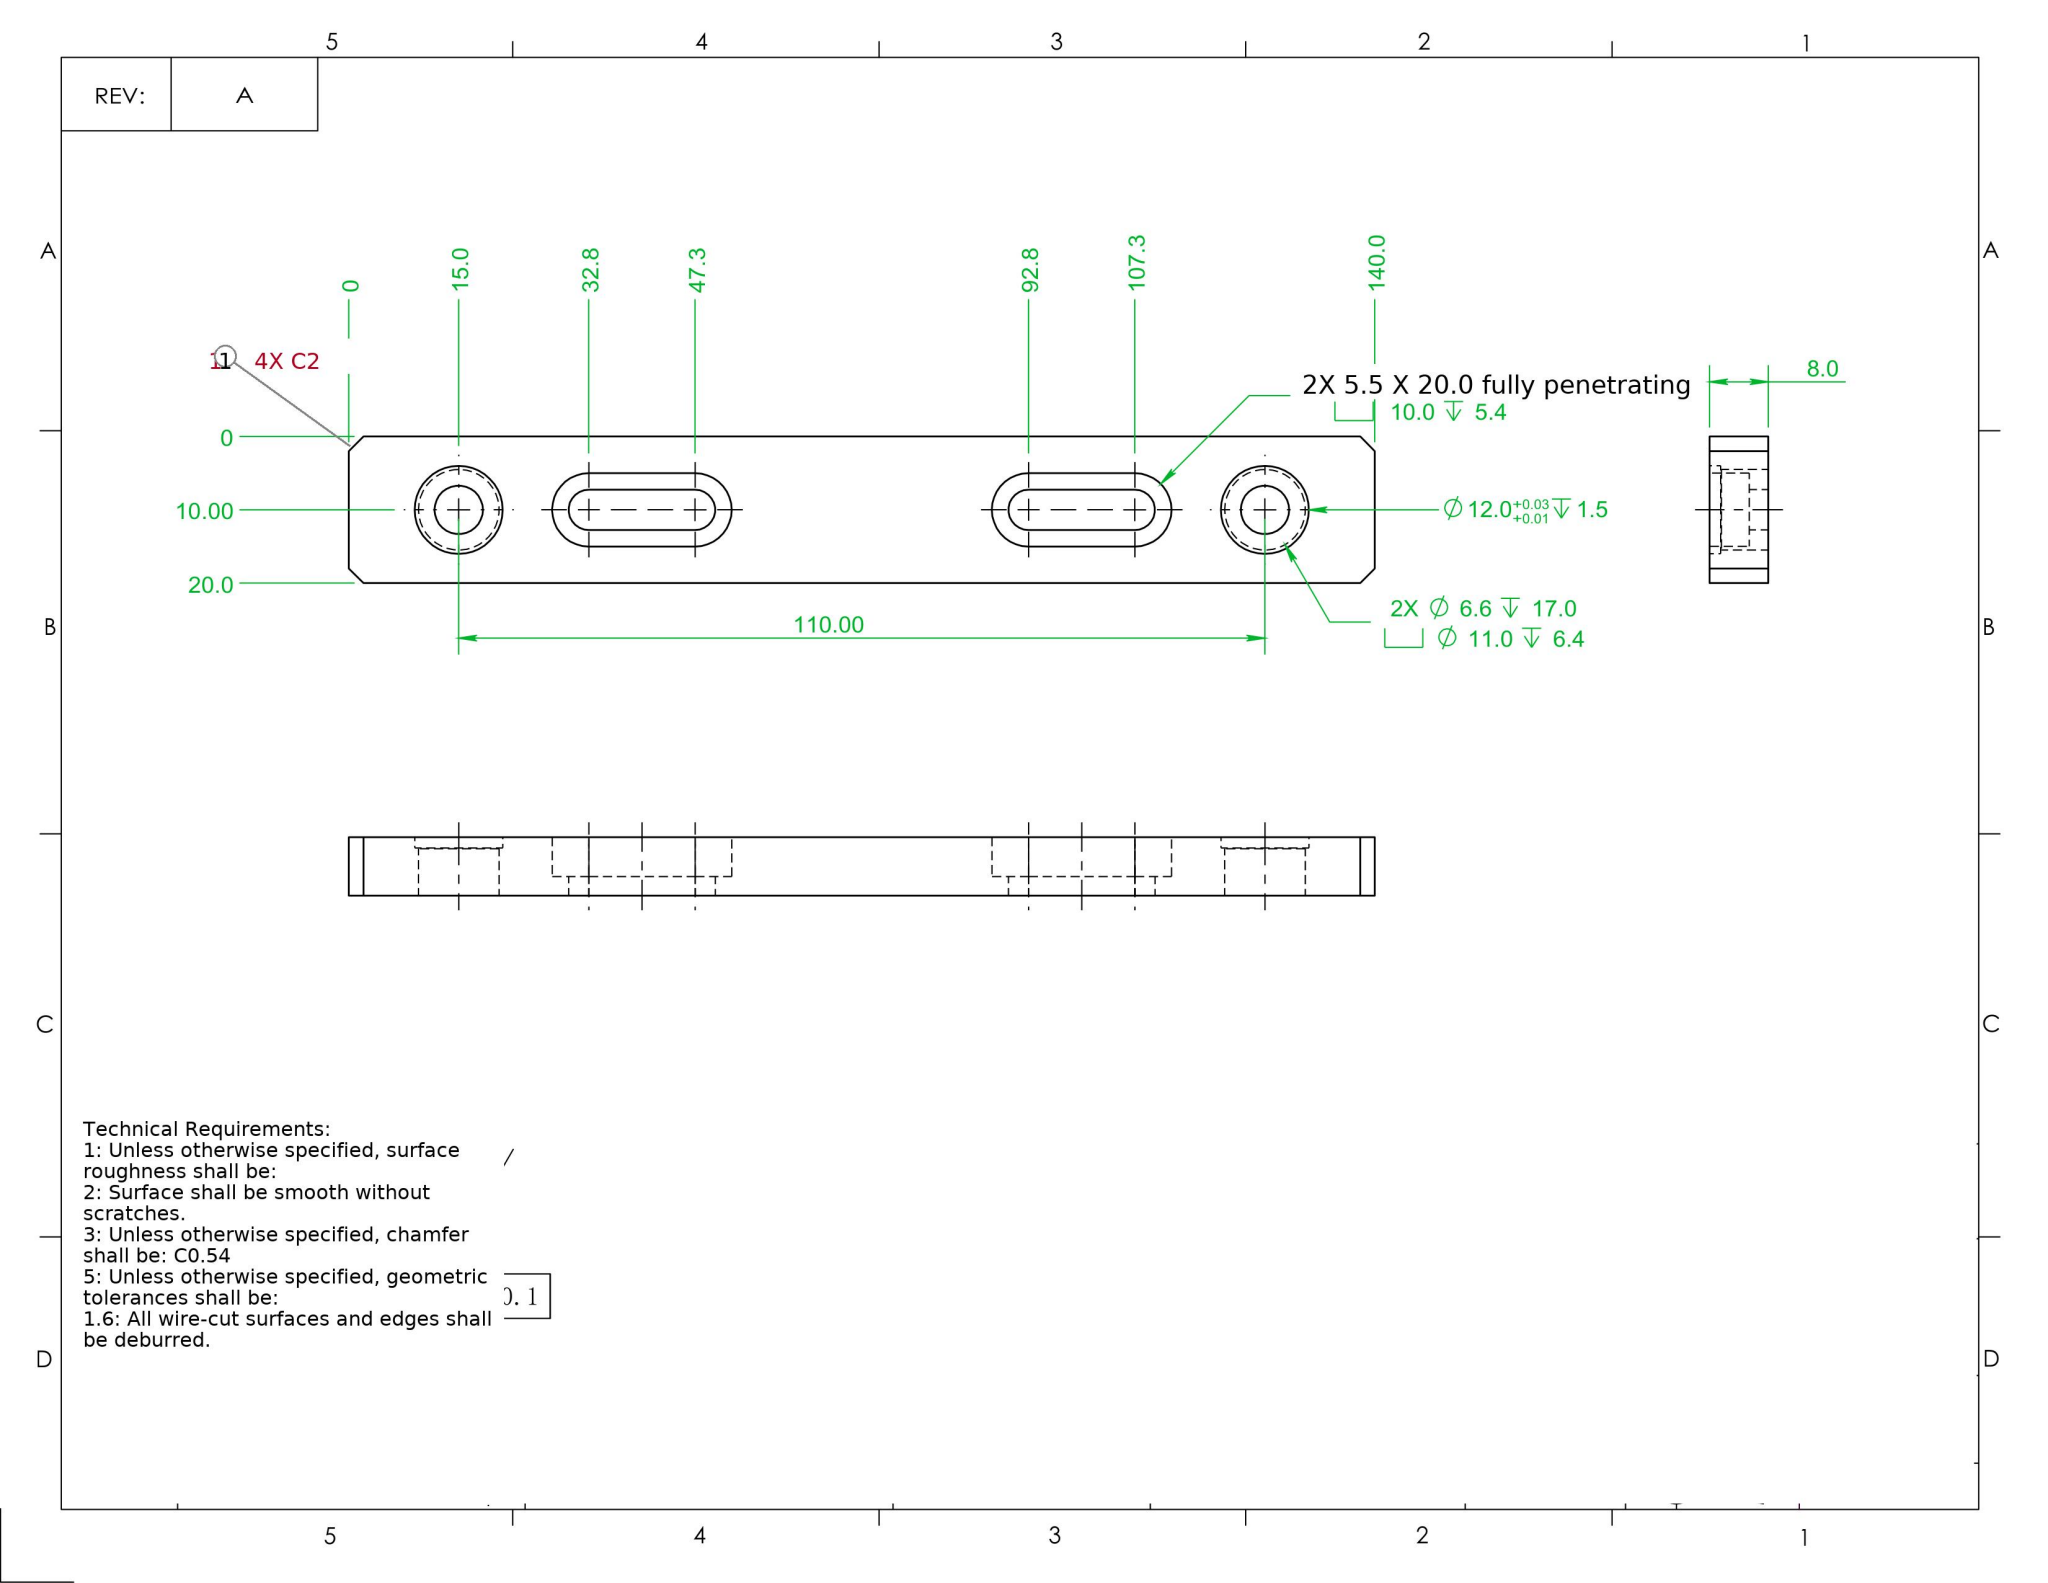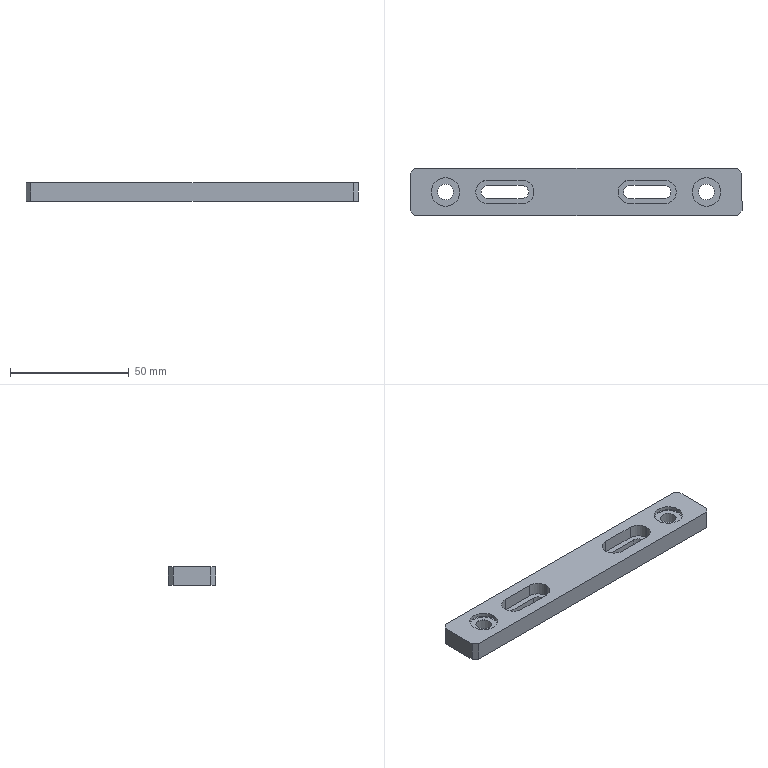Part | SolidWorks | mm | 1 solid | 48 faces | box 140 x 20 x 8 mm | volume 17821 mm3 | cylinder 24 | plane 24 | commonest cylinder face diameters 10 x6 5.5 x6 11 x4 6.6 x4 12 x4